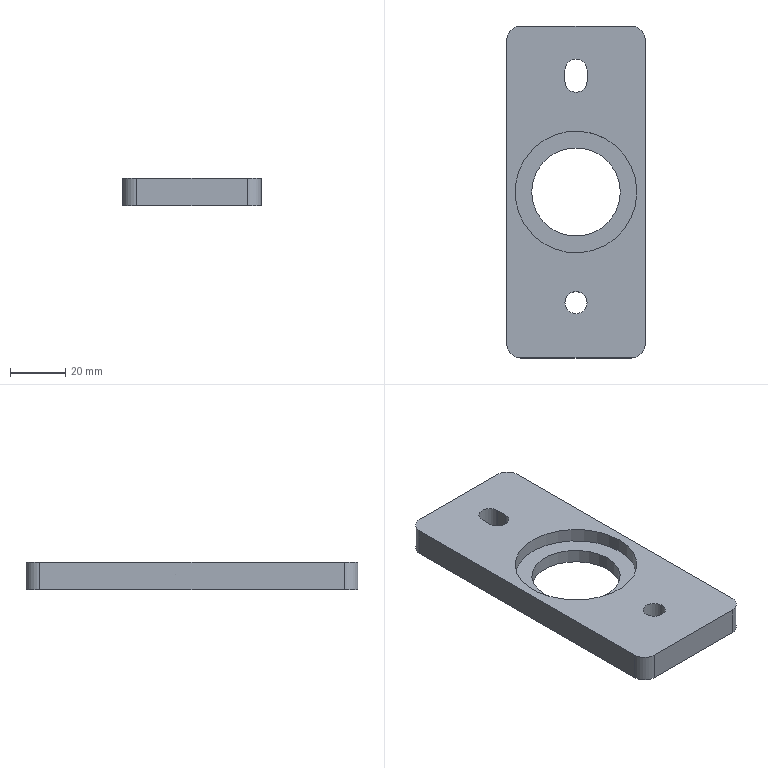Component | NX | CLAMP_PLATE | 1 solid | 18 faces | volume 46836 mm3 | cylinder 9 | plane 9 | commonest cylinder face diameters 10 x4 8 x3 32 x1 44 x1